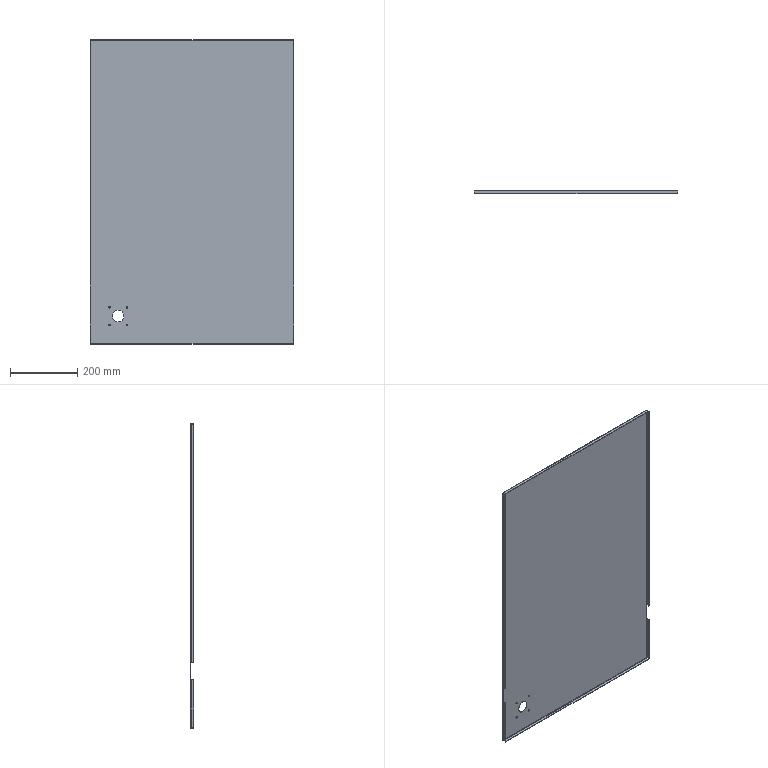Component | SolidWorks | UpperDoorFrame-1_TopPlate-1 | 1 solid | 60 faces | volume 858514 mm3 | plane 32 | cylinder 20 | spline 8 | commonest cylinder face diameters 4.2 x8 1.473 x6 4.473 x4 34.641 x2